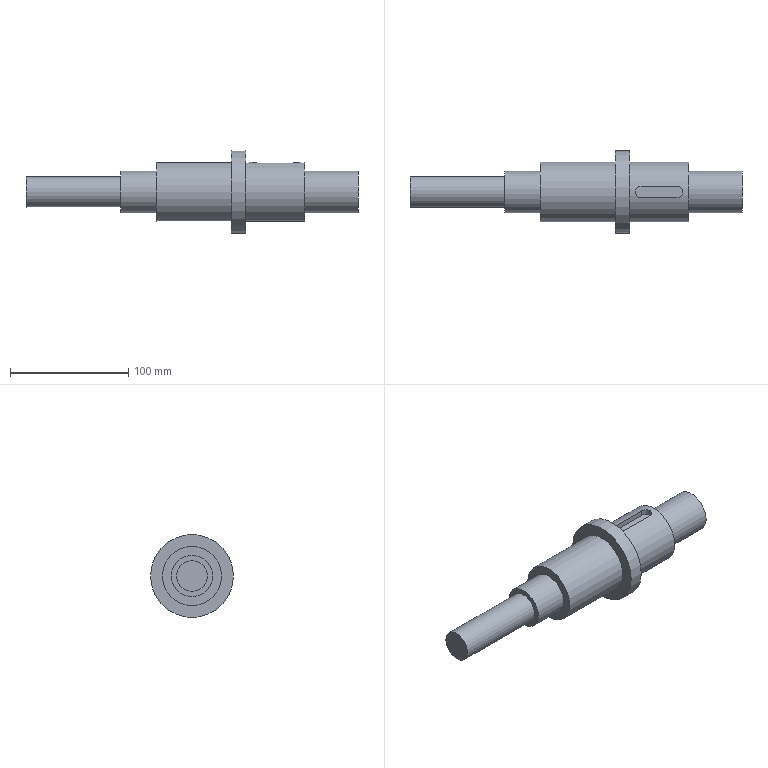Component | NX | SHUCHUZHOU | 1 solid | 18 faces | box 280.5 x 70 x 70 mm | volume 381839 mm3 | plane 10 | cylinder 8 | commonest cylinder face diameters 50 x2 35 x2 10 x2 70 x1 26 x1
STEP:
#1=CARTESIAN_POINT('',(0.,0.,0.));
#2=DIRECTION('',(0.,0.,1.));
#3=DIRECTION('',(1.,0.,0.));
#4=AXIS2_PLACEMENT_3D('',#1,#2,#3);
#5=CARTESIAN_POINT('',(5.25,225.,-88.));
#6=VERTEX_POINT('',#5);
#7=CARTESIAN_POINT('',(5.25,200.,-88.));
#8=DIRECTION('',(1.,0.,0.));
#9=DIRECTION('',(0.,1.,0.));
#10=AXIS2_PLACEMENT_3D('',#7,#8,#9);
#11=CIRCLE('',#10,25.);
#12=CARTESIAN_POINT('',(55.25,200.,-88.));
#13=DIRECTION('',(-1.,0.,0.));
#14=DIRECTION('',(0.,0.,1.));
#15=AXIS2_PLACEMENT_3D('',#12,#13,#14);
#16=CYLINDRICAL_SURFACE('',#15,25.);
#17=CARTESIAN_POINT('',(7.854,50.));
#18=DIRECTION('',(-1.,0.));
#19=VECTOR('',#18,1.);
#20=LINE('',#17,#19);
#21=(GEOMETRIC_REPRESENTATION_CONTEXT(2)PARAMETRIC_REPRESENTATION_CONTEXT()REPRESENTATION_CONTEXT('',''));
#22=DEFINITIONAL_REPRESENTATION('',(#20),#21);
#23=PCURVE('',#16,#22);
#24=CARTESIAN_POINT('',(5.25,200.,-88.));
#25=DIRECTION('',(1.,0.,0.));
#26=DIRECTION('',(0.,0.,-1.));
#27=AXIS2_PLACEMENT_3D('',#24,#25,#26);
#28=PLANE('',#27);
#29=CARTESIAN_POINT('',(0.,0.));
#30=DIRECTION('',(0.,1.));
#31=AXIS2_PLACEMENT_2D('',#29,#30);
#32=CIRCLE('',#31,25.);
#33=(GEOMETRIC_REPRESENTATION_CONTEXT(2)PARAMETRIC_REPRESENTATION_CONTEXT()REPRESENTATION_CONTEXT('',''));
#34=DEFINITIONAL_REPRESENTATION('',(#32),#33);
#35=PCURVE('',#28,#34);
#36=SURFACE_CURVE('',#11,(#23,#35),.PCURVE_S1.);
#37=EDGE_CURVE('',#6,#6,#36,.T.);
#38=ORIENTED_EDGE('',*,*,#37,.T.);
#39=CARTESIAN_POINT('',(55.25,225.,-88.));
#40=VERTEX_POINT('',#39);
#41=CARTESIAN_POINT('',(55.25,225.,-88.));
#42=CARTESIAN_POINT('',(5.25,225.,-88.));
#43=B_SPLINE_CURVE_WITH_KNOTS('',1,(#41,#42),.UNSPECIFIED.,.F.,.F.,(2,2),(0.,50.),.PIECEWISE_BEZIER_KNOTS.);
#44=CARTESIAN_POINT('',(1.571,0.));
#45=DIRECTION('',(0.,1.));
#46=VECTOR('',#45,1.);
#47=LINE('',#44,#46);
#48=(GEOMETRIC_REPRESENTATION_CONTEXT(2)PARAMETRIC_REPRESENTATION_CONTEXT()REPRESENTATION_CONTEXT('',''));
#49=DEFINITIONAL_REPRESENTATION('',(#47),#48);
#50=PCURVE('',#16,#49);
#51=CARTESIAN_POINT('',(7.854,0.));
#52=DIRECTION('',(0.,1.));
#53=VECTOR('',#52,1.);
#54=LINE('',#51,#53);
#55=(GEOMETRIC_REPRESENTATION_CONTEXT(2)PARAMETRIC_REPRESENTATION_CONTEXT()REPRESENTATION_CONTEXT('',''));
#56=DEFINITIONAL_REPRESENTATION('',(#54),#55);
#57=PCURVE('',#16,#56);
#58=SEAM_CURVE('',#43,(#50,#57),.PCURVE_S1.);
#59=EDGE_CURVE('',#40,#6,#58,.T.);
#60=ORIENTED_EDGE('',*,*,#59,.F.);
#61=CARTESIAN_POINT('',(55.25,200.,-88.));
#62=DIRECTION('',(1.,0.,0.));
#63=DIRECTION('',(0.,1.,0.));
#64=AXIS2_PLACEMENT_3D('',#61,#62,#63);
#65=CIRCLE('',#64,25.);
#66=CARTESIAN_POINT('',(7.854,0.));
#67=DIRECTION('',(-1.,0.));
#68=VECTOR('',#67,1.);
#69=LINE('',#66,#68);
#70=(GEOMETRIC_REPRESENTATION_CONTEXT(2)PARAMETRIC_REPRESENTATION_CONTEXT()REPRESENTATION_CONTEXT('',''));
#71=DEFINITIONAL_REPRESENTATION('',(#69),#70);
#72=PCURVE('',#16,#71);
#73=CARTESIAN_POINT('',(55.25,200.,-88.));
#74=DIRECTION('',(1.,0.,0.));
#75=DIRECTION('',(0.,0.,-1.));
#76=AXIS2_PLACEMENT_3D('',#73,#74,#75);
#77=PLANE('',#76);
#78=CARTESIAN_POINT('',(0.,0.));
#79=DIRECTION('',(0.,1.));
#80=AXIS2_PLACEMENT_2D('',#78,#79);
#81=CIRCLE('',#80,25.);
#82=(GEOMETRIC_REPRESENTATION_CONTEXT(2)PARAMETRIC_REPRESENTATION_CONTEXT()REPRESENTATION_CONTEXT('',''));
#83=DEFINITIONAL_REPRESENTATION('',(#81),#82);
#84=PCURVE('',#77,#83);
#85=SURFACE_CURVE('',#65,(#72,#84),.PCURVE_S1.);
#86=EDGE_CURVE('',#40,#40,#85,.T.);
#87=ORIENTED_EDGE('',*,*,#86,.F.);
#88=ORIENTED_EDGE('',*,*,#59,.T.);
#89=EDGE_LOOP('',(#38,#60,#87,#88));
#90=FACE_BOUND('',#89,.T.);
#91=CARTESIAN_POINT('',(15.25,205.,-63.505));
#92=VERTEX_POINT('',#91);
#93=CARTESIAN_POINT('',(15.25,195.,-63.505));
#94=VERTEX_POINT('',#93);
#95=CARTESIAN_POINT('',(15.25,205.,-63.505));
#96=CARTESIAN_POINT('',(13.925,205.,-63.505));
#97=CARTESIAN_POINT('',(12.634,204.455,-63.383));
#98=CARTESIAN_POINT('',(10.795,202.616,-63.12));
#99=CARTESIAN_POINT('',(10.251,201.312,-63.));
#100=CARTESIAN_POINT('',(10.249,198.696,-63.));
#101=CARTESIAN_POINT('',(10.784,197.396,-63.118));
#102=CARTESIAN_POINT('',(12.641,195.536,-63.384));
#103=CARTESIAN_POINT('',(13.925,195.,-63.505));
#104=CARTESIAN_POINT('',(15.25,195.,-63.505));
#105=B_SPLINE_CURVE_WITH_KNOTS('',3,(#95,#96,#97,#98,#99,#100,#101,#102,#103,#104),.UNSPECIFIED.,.F.,.F.,(4,2,2,2,4),(0.,0.25,0.5,0.75,1.),.UNSPECIFIED.);
#106=CARTESIAN_POINT('',(6.485,40.));
#107=CARTESIAN_POINT('',(6.485,40.241));
#108=CARTESIAN_POINT('',(6.483,40.72));
#109=CARTESIAN_POINT('',(6.477,41.421));
#110=CARTESIAN_POINT('',(6.466,42.09));
#111=CARTESIAN_POINT('',(6.453,42.716));
#112=CARTESIAN_POINT('',(6.435,43.287));
#113=CARTESIAN_POINT('',(6.415,43.79));
#114=CARTESIAN_POINT('',(6.392,44.215));
#115=CARTESIAN_POINT('',(6.367,44.556));
#116=CARTESIAN_POINT('',(6.34,44.808));
#117=CARTESIAN_POINT('',(6.312,44.964));
#118=CARTESIAN_POINT('',(6.283,45.018));
#119=CARTESIAN_POINT('',(6.255,44.965));
#120=CARTESIAN_POINT('',(6.227,44.811));
#121=CARTESIAN_POINT('',(6.2,44.562));
#122=CARTESIAN_POINT('',(6.175,44.221));
#123=CARTESIAN_POINT('',(6.152,43.794));
#124=CARTESIAN_POINT('',(6.131,43.286));
#125=CARTESIAN_POINT('',(6.114,42.713));
#126=CARTESIAN_POINT('',(6.1,42.087));
#127=CARTESIAN_POINT('',(6.09,41.419));
#128=CARTESIAN_POINT('',(6.083,40.72));
#129=CARTESIAN_POINT('',(6.082,40.241));
#130=CARTESIAN_POINT('',(6.082,40.));
#131=B_SPLINE_CURVE_WITH_KNOTS('',3,(#106,#107,#108,#109,#110,#111,#112,#113,#114,#115,#116,#117,#118,#119,#120,#121,#122,#123,#124,#125,#126,#127,#128,#129,#130),.UNSPECIFIED.,.F.,.F.,(4,1,1,1,1,1,1,1,1,1,1,1,1,1,1,1,1,1,1,1,1,1,4),(0.,0.04545,0.09091,0.1364,0.1818,0.2273,0.2727,0.3182,0.3636,0.4091,0.4545,0.5,0.5455,0.5909,0.6364,0.6818,0.7273,0.7727,0.8182,0.8636,0.9091,0.9545,1.),.QUASI_UNIFORM_KNOTS.);
#132=(GEOMETRIC_REPRESENTATION_CONTEXT(2)PARAMETRIC_REPRESENTATION_CONTEXT()REPRESENTATION_CONTEXT('',''));
#133=DEFINITIONAL_REPRESENTATION('',(#131),#132);
#134=PCURVE('',#16,#133);
#135=CARTESIAN_POINT('',(15.25,200.,-27.));
#136=DIRECTION('',(0.,0.,-1.));
#137=DIRECTION('',(-1.,0.,0.));
#138=AXIS2_PLACEMENT_3D('',#135,#136,#137);
#139=CYLINDRICAL_SURFACE('',#138,5.);
#140=CARTESIAN_POINT('',(1.571,36.505));
#141=CARTESIAN_POINT('',(1.523,36.505));
#142=CARTESIAN_POINT('',(1.427,36.497));
#143=CARTESIAN_POINT('',(1.284,36.465));
#144=CARTESIAN_POINT('',(1.141,36.416));
#145=CARTESIAN_POINT('',(0.9983,36.356));
#146=CARTESIAN_POINT('',(0.8563,36.287));
#147=CARTESIAN_POINT('',(0.7145,36.215));
#148=CARTESIAN_POINT('',(0.5722,36.147));
#149=CARTESIAN_POINT('',(0.4294,36.087));
#150=CARTESIAN_POINT('',(0.2863,36.04));
#151=CARTESIAN_POINT('',(0.1435,36.008));
#152=CARTESIAN_POINT('',(0.0007954,35.996));
#153=CARTESIAN_POINT('',(-0.1418,36.008));
#154=CARTESIAN_POINT('',(-0.2844,36.039));
#155=CARTESIAN_POINT('',(-0.4273,36.087));
#156=CARTESIAN_POINT('',(-0.5702,36.146));
#157=CARTESIAN_POINT('',(-0.7132,36.214));
#158=CARTESIAN_POINT('',(-0.8566,36.288));
#159=CARTESIAN_POINT('',(-0.9991,36.356));
#160=CARTESIAN_POINT('',(-1.141,36.417));
#161=CARTESIAN_POINT('',(-1.284,36.465));
#162=CARTESIAN_POINT('',(-1.427,36.497));
#163=CARTESIAN_POINT('',(-1.523,36.505));
#164=CARTESIAN_POINT('',(-1.571,36.505));
#165=B_SPLINE_CURVE_WITH_KNOTS('',3,(#140,#141,#142,#143,#144,#145,#146,#147,#148,#149,#150,#151,#152,#153,#154,#155,#156,#157,#158,#159,#160,#161,#162,#163,#164),.UNSPECIFIED.,.F.,.F.,(4,1,1,1,1,1,1,1,1,1,1,1,1,1,1,1,1,1,1,1,1,1,4),(0.,0.04545,0.09091,0.1364,0.1818,0.2273,0.2727,0.3182,0.3636,0.4091,0.4545,0.5,0.5455,0.5909,0.6364,0.6818,0.7273,0.7727,0.8182,0.8636,0.9091,0.9545,1.),.QUASI_UNIFORM_KNOTS.);
#166=(GEOMETRIC_REPRESENTATION_CONTEXT(2)PARAMETRIC_REPRESENTATION_CONTEXT()REPRESENTATION_CONTEXT('',''));
#167=DEFINITIONAL_REPRESENTATION('',(#165),#166);
#168=PCURVE('',#139,#167);
#169=SURFACE_CURVE('',#105,(#134,#168),.PCURVE_S1.);
#170=EDGE_CURVE('',#92,#94,#169,.T.);
#171=ORIENTED_EDGE('',*,*,#170,.F.);
#172=CARTESIAN_POINT('',(45.25,205.,-63.505));
#173=VERTEX_POINT('',#172);
#174=CARTESIAN_POINT('',(55.25,205.,-63.505));
#175=DIRECTION('',(-1.,0.,0.));
#176=VECTOR('',#175,1.);
#177=LINE('',#174,#176);
#178=CARTESIAN_POINT('',(6.485,0.));
#179=DIRECTION('',(0.,1.));
#180=VECTOR('',#179,1.);
#181=LINE('',#178,#180);
#182=(GEOMETRIC_REPRESENTATION_CONTEXT(2)PARAMETRIC_REPRESENTATION_CONTEXT()REPRESENTATION_CONTEXT('',''));
#183=DEFINITIONAL_REPRESENTATION('',(#181),#182);
#184=PCURVE('',#16,#183);
#185=CARTESIAN_POINT('',(45.25,205.,-27.));
#186=DIRECTION('',(0.,-1.,0.));
#187=DIRECTION('',(0.,0.,-1.));
#188=AXIS2_PLACEMENT_3D('',#185,#186,#187);
#189=PLANE('',#188);
#190=CARTESIAN_POINT('',(36.505,10.));
#191=DIRECTION('',(0.,-1.));
#192=VECTOR('',#191,1.);
#193=LINE('',#190,#192);
#194=(GEOMETRIC_REPRESENTATION_CONTEXT(2)PARAMETRIC_REPRESENTATION_CONTEXT()REPRESENTATION_CONTEXT('',''));
#195=DEFINITIONAL_REPRESENTATION('',(#193),#194);
#196=PCURVE('',#189,#195);
#197=SURFACE_CURVE('',#177,(#184,#196),.PCURVE_S1.);
#198=EDGE_CURVE('',#173,#92,#197,.T.);
#199=ORIENTED_EDGE('',*,*,#198,.F.);
#200=CARTESIAN_POINT('',(45.25,195.,-63.505));
#201=VERTEX_POINT('',#200);
#202=CARTESIAN_POINT('',(45.25,195.,-63.505));
#203=CARTESIAN_POINT('',(46.575,195.,-63.505));
#204=CARTESIAN_POINT('',(47.866,195.545,-63.383));
#205=CARTESIAN_POINT('',(49.705,197.384,-63.12));
#206=CARTESIAN_POINT('',(50.249,198.688,-63.));
#207=CARTESIAN_POINT('',(50.251,201.304,-63.));
#208=CARTESIAN_POINT('',(49.716,202.604,-63.118));
#209=CARTESIAN_POINT('',(47.859,204.464,-63.384));
#210=CARTESIAN_POINT('',(46.575,205.,-63.505));
#211=CARTESIAN_POINT('',(45.25,205.,-63.505));
#212=B_SPLINE_CURVE_WITH_KNOTS('',3,(#202,#203,#204,#205,#206,#207,#208,#209,#210,#211),.UNSPECIFIED.,.F.,.F.,(4,2,2,2,4),(0.,0.25,0.5,0.75,1.),.UNSPECIFIED.);
#213=CARTESIAN_POINT('',(6.082,10.));
#214=CARTESIAN_POINT('',(6.082,9.759));
#215=CARTESIAN_POINT('',(6.083,9.28));
#216=CARTESIAN_POINT('',(6.09,8.579));
#217=CARTESIAN_POINT('',(6.1,7.91));
#218=CARTESIAN_POINT('',(6.114,7.284));
#219=CARTESIAN_POINT('',(6.131,6.713));
#220=CARTESIAN_POINT('',(6.151,6.21));
#221=CARTESIAN_POINT('',(6.174,5.785));
#222=CARTESIAN_POINT('',(6.2,5.444));
#223=CARTESIAN_POINT('',(6.227,5.192));
#224=CARTESIAN_POINT('',(6.254,5.036));
#225=CARTESIAN_POINT('',(6.283,4.982));
#226=CARTESIAN_POINT('',(6.312,5.035));
#227=CARTESIAN_POINT('',(6.339,5.189));
#228=CARTESIAN_POINT('',(6.366,5.438));
#229=CARTESIAN_POINT('',(6.392,5.779));
#230=CARTESIAN_POINT('',(6.415,6.206));
#231=CARTESIAN_POINT('',(6.435,6.714));
#232=CARTESIAN_POINT('',(6.453,7.287));
#233=CARTESIAN_POINT('',(6.467,7.913));
#234=CARTESIAN_POINT('',(6.477,8.581));
#235=CARTESIAN_POINT('',(6.483,9.28));
#236=CARTESIAN_POINT('',(6.485,9.759));
#237=CARTESIAN_POINT('',(6.485,10.));
#238=B_SPLINE_CURVE_WITH_KNOTS('',3,(#213,#214,#215,#216,#217,#218,#219,#220,#221,#222,#223,#224,#225,#226,#227,#228,#229,#230,#231,#232,#233,#234,#235,#236,#237),.UNSPECIFIED.,.F.,.F.,(4,1,1,1,1,1,1,1,1,1,1,1,1,1,1,1,1,1,1,1,1,1,4),(0.,0.04545,0.09091,0.1364,0.1818,0.2273,0.2727,0.3182,0.3636,0.4091,0.4545,0.5,0.5455,0.5909,0.6364,0.6818,0.7273,0.7727,0.8182,0.8636,0.9091,0.9545,1.),.QUASI_UNIFORM_KNOTS.);
#239=(GEOMETRIC_REPRESENTATION_CONTEXT(2)PARAMETRIC_REPRESENTATION_CONTEXT()REPRESENTATION_CONTEXT('',''));
#240=DEFINITIONAL_REPRESENTATION('',(#238),#239);
#241=PCURVE('',#16,#240);
#242=CARTESIAN_POINT('',(45.25,200.,-27.));
#243=DIRECTION('',(0.,0.,-1.));
#244=DIRECTION('',(-1.,0.,0.));
#245=AXIS2_PLACEMENT_3D('',#242,#243,#244);
#246=CYLINDRICAL_SURFACE('',#245,5.);
#247=CARTESIAN_POINT('',(4.712,36.505));
#248=CARTESIAN_POINT('',(4.664,36.505));
#249=CARTESIAN_POINT('',(4.568,36.497));
#250=CARTESIAN_POINT('',(4.425,36.465));
#251=CARTESIAN_POINT('',(4.282,36.416));
#252=CARTESIAN_POINT('',(4.14,36.356));
#253=CARTESIAN_POINT('',(3.998,36.287));
#254=CARTESIAN_POINT('',(3.856,36.215));
#255=CARTESIAN_POINT('',(3.714,36.147));
#256=CARTESIAN_POINT('',(3.571,36.087));
#257=CARTESIAN_POINT('',(3.428,36.04));
#258=CARTESIAN_POINT('',(3.285,36.008));
#259=CARTESIAN_POINT('',(3.142,35.996));
#260=CARTESIAN_POINT('',(3.,36.008));
#261=CARTESIAN_POINT('',(2.857,36.039));
#262=CARTESIAN_POINT('',(2.714,36.087));
#263=CARTESIAN_POINT('',(2.571,36.146));
#264=CARTESIAN_POINT('',(2.428,36.214));
#265=CARTESIAN_POINT('',(2.285,36.288));
#266=CARTESIAN_POINT('',(2.142,36.356));
#267=CARTESIAN_POINT('',(2.,36.417));
#268=CARTESIAN_POINT('',(1.858,36.465));
#269=CARTESIAN_POINT('',(1.715,36.497));
#270=CARTESIAN_POINT('',(1.619,36.505));
#271=CARTESIAN_POINT('',(1.571,36.505));
#272=B_SPLINE_CURVE_WITH_KNOTS('',3,(#247,#248,#249,#250,#251,#252,#253,#254,#255,#256,#257,#258,#259,#260,#261,#262,#263,#264,#265,#266,#267,#268,#269,#270,#271),.UNSPECIFIED.,.F.,.F.,(4,1,1,1,1,1,1,1,1,1,1,1,1,1,1,1,1,1,1,1,1,1,4),(0.,0.04545,0.09091,0.1364,0.1818,0.2273,0.2727,0.3182,0.3636,0.4091,0.4545,0.5,0.5455,0.5909,0.6364,0.6818,0.7273,0.7727,0.8182,0.8636,0.9091,0.9545,1.),.QUASI_UNIFORM_KNOTS.);
#273=(GEOMETRIC_REPRESENTATION_CONTEXT(2)PARAMETRIC_REPRESENTATION_CONTEXT()REPRESENTATION_CONTEXT('',''));
#274=DEFINITIONAL_REPRESENTATION('',(#272),#273);
#275=PCURVE('',#246,#274);
#276=SURFACE_CURVE('',#212,(#241,#275),.PCURVE_S1.);
#277=EDGE_CURVE('',#201,#173,#276,.T.);
#278=ORIENTED_EDGE('',*,*,#277,.F.);
#279=CARTESIAN_POINT('',(55.25,195.,-63.505));
#280=DIRECTION('',(1.,0.,0.));
#281=VECTOR('',#280,1.);
#282=LINE('',#279,#281);
#283=CARTESIAN_POINT('',(6.082,0.));
#284=DIRECTION('',(0.,-1.));
#285=VECTOR('',#284,1.);
#286=LINE('',#283,#285);
#287=(GEOMETRIC_REPRESENTATION_CONTEXT(2)PARAMETRIC_REPRESENTATION_CONTEXT()REPRESENTATION_CONTEXT('',''));
#288=DEFINITIONAL_REPRESENTATION('',(#286),#287);
#289=PCURVE('',#16,#288);
#290=CARTESIAN_POINT('',(15.25,195.,-27.));
#291=DIRECTION('',(-0.,1.,0.));
#292=DIRECTION('',(-1.,-0.,0.));
#293=AXIS2_PLACEMENT_3D('',#290,#291,#292);
#294=PLANE('',#293);
#295=CARTESIAN_POINT('',(-40.,-36.505));
#296=DIRECTION('',(-1.,0.));
#297=VECTOR('',#296,1.);
#298=LINE('',#295,#297);
#299=(GEOMETRIC_REPRESENTATION_CONTEXT(2)PARAMETRIC_REPRESENTATION_CONTEXT()REPRESENTATION_CONTEXT('',''));
#300=DEFINITIONAL_REPRESENTATION('',(#298),#299);
#301=PCURVE('',#294,#300);
#302=SURFACE_CURVE('',#282,(#289,#301),.PCURVE_S1.);
#303=EDGE_CURVE('',#94,#201,#302,.T.);
#304=ORIENTED_EDGE('',*,*,#303,.F.);
#305=EDGE_LOOP('',(#171,#199,#278,#304));
#306=FACE_BOUND('',#305,.T.);
#307=ADVANCED_FACE('',(#90,#306),#16,.T.);
#308=CARTESIAN_POINT('',(-6.75,235.,-88.));
#309=VERTEX_POINT('',#308);
#310=CARTESIAN_POINT('',(-6.75,200.,-88.));
#311=DIRECTION('',(1.,0.,0.));
#312=DIRECTION('',(0.,1.,0.));
#313=AXIS2_PLACEMENT_3D('',#310,#311,#312);
#314=CIRCLE('',#313,35.);
#315=CARTESIAN_POINT('',(-6.75,200.,-88.));
#316=DIRECTION('',(1.,0.,0.));
#317=DIRECTION('',(0.,0.,-1.));
#318=AXIS2_PLACEMENT_3D('',#315,#316,#317);
#319=PLANE('',#318);
#320=CARTESIAN_POINT('',(0.,0.));
#321=DIRECTION('',(0.,1.));
#322=AXIS2_PLACEMENT_2D('',#320,#321);
#323=CIRCLE('',#322,35.);
#324=(GEOMETRIC_REPRESENTATION_CONTEXT(2)PARAMETRIC_REPRESENTATION_CONTEXT()REPRESENTATION_CONTEXT('',''));
#325=DEFINITIONAL_REPRESENTATION('',(#323),#324);
#326=PCURVE('',#319,#325);
#327=CARTESIAN_POINT('',(5.25,200.,-88.));
#328=DIRECTION('',(-1.,0.,0.));
#329=DIRECTION('',(0.,0.,1.));
#330=AXIS2_PLACEMENT_3D('',#327,#328,#329);
#331=CYLINDRICAL_SURFACE('',#330,35.);
#332=CARTESIAN_POINT('',(7.854,12.));
#333=DIRECTION('',(-1.,0.));
#334=VECTOR('',#333,1.);
#335=LINE('',#332,#334);
#336=(GEOMETRIC_REPRESENTATION_CONTEXT(2)PARAMETRIC_REPRESENTATION_CONTEXT()REPRESENTATION_CONTEXT('',''));
#337=DEFINITIONAL_REPRESENTATION('',(#335),#336);
#338=PCURVE('',#331,#337);
#339=SURFACE_CURVE('',#314,(#326,#338),.PCURVE_S1.);
#340=EDGE_CURVE('',#309,#309,#339,.T.);
#341=ORIENTED_EDGE('',*,*,#340,.F.);
#342=EDGE_LOOP('',(#341));
#343=FACE_BOUND('',#342,.T.);
#344=CARTESIAN_POINT('',(-6.75,225.,-88.));
#345=VERTEX_POINT('',#344);
#346=CARTESIAN_POINT('',(-6.75,200.,-88.));
#347=DIRECTION('',(-1.,0.,0.));
#348=DIRECTION('',(0.,1.,0.));
#349=AXIS2_PLACEMENT_3D('',#346,#347,#348);
#350=CIRCLE('',#349,25.);
#351=CARTESIAN_POINT('',(0.,25.));
#352=CARTESIAN_POINT('',(43.301,25.));
#353=CARTESIAN_POINT('',(21.651,-12.5));
#354=CARTESIAN_POINT('',(0.,-50.));
#355=CARTESIAN_POINT('',(-21.651,-12.5));
#356=CARTESIAN_POINT('',(-43.301,25.));
#357=CARTESIAN_POINT('',(0.,25.));
#358=(BOUNDED_CURVE()B_SPLINE_CURVE(2,(#351,#352,#353,#354,#355,#356,#357),.UNSPECIFIED.,.T.,.F.)B_SPLINE_CURVE_WITH_KNOTS((1,2,2,2,2,1),(-2.094,0.,2.094,4.189,6.283,8.378),.UNSPECIFIED.)CURVE()GEOMETRIC_REPRESENTATION_ITEM()RATIONAL_B_SPLINE_CURVE((1.,0.5,1.,0.5,1.,0.5,1.))REPRESENTATION_ITEM(''));
#359=(GEOMETRIC_REPRESENTATION_CONTEXT(2)PARAMETRIC_REPRESENTATION_CONTEXT()REPRESENTATION_CONTEXT('',''));
#360=DEFINITIONAL_REPRESENTATION('',(#358),#359);
#361=PCURVE('',#319,#360);
#362=CARTESIAN_POINT('',(-70.25,200.,-88.));
#363=DIRECTION('',(1.,0.,0.));
#364=DIRECTION('',(0.,0.,-1.));
#365=AXIS2_PLACEMENT_3D('',#362,#363,#364);
#366=CYLINDRICAL_SURFACE('',#365,25.);
#367=CARTESIAN_POINT('',(7.854,63.5));
#368=DIRECTION('',(-1.,0.));
#369=VECTOR('',#368,1.);
#370=LINE('',#367,#369);
#371=(GEOMETRIC_REPRESENTATION_CONTEXT(2)PARAMETRIC_REPRESENTATION_CONTEXT()REPRESENTATION_CONTEXT('',''));
#372=DEFINITIONAL_REPRESENTATION('',(#370),#371);
#373=PCURVE('',#366,#372);
#374=SURFACE_CURVE('',#350,(#361,#373),.PCURVE_S1.);
#375=EDGE_CURVE('',#345,#345,#374,.T.);
#376=ORIENTED_EDGE('',*,*,#375,.F.);
#377=EDGE_LOOP('',(#376));
#378=FACE_BOUND('',#377,.T.);
#379=ADVANCED_FACE('',(#343,#378),#319,.F.);
#380=CARTESIAN_POINT('',(5.25,235.,-88.));
#381=VERTEX_POINT('',#380);
#382=CARTESIAN_POINT('',(5.25,200.,-88.));
#383=DIRECTION('',(1.,0.,0.));
#384=DIRECTION('',(0.,1.,0.));
#385=AXIS2_PLACEMENT_3D('',#382,#383,#384);
#386=CIRCLE('',#385,35.);
#387=CARTESIAN_POINT('',(7.854,0.));
#388=DIRECTION('',(-1.,0.));
#389=VECTOR('',#388,1.);
#390=LINE('',#387,#389);
#391=(GEOMETRIC_REPRESENTATION_CONTEXT(2)PARAMETRIC_REPRESENTATION_CONTEXT()REPRESENTATION_CONTEXT('',''));
#392=DEFINITIONAL_REPRESENTATION('',(#390),#391);
#393=PCURVE('',#331,#392);
#394=CARTESIAN_POINT('',(0.,0.));
#395=DIRECTION('',(0.,1.));
#396=AXIS2_PLACEMENT_2D('',#394,#395);
#397=CIRCLE('',#396,35.);
#398=(GEOMETRIC_REPRESENTATION_CONTEXT(2)PARAMETRIC_REPRESENTATION_CONTEXT()REPRESENTATION_CONTEXT('',''));
#399=DEFINITIONAL_REPRESENTATION('',(#397),#398);
#400=PCURVE('',#28,#399);
#401=SURFACE_CURVE('',#386,(#393,#400),.PCURVE_S1.);
#402=EDGE_CURVE('',#381,#381,#401,.T.);
#403=ORIENTED_EDGE('',*,*,#402,.F.);
#404=CARTESIAN_POINT('',(5.25,235.,-88.));
#405=CARTESIAN_POINT('',(-6.75,235.,-88.));
#406=B_SPLINE_CURVE_WITH_KNOTS('',1,(#404,#405),.UNSPECIFIED.,.F.,.F.,(2,2),(0.,12.),.PIECEWISE_BEZIER_KNOTS.);
#407=CARTESIAN_POINT('',(7.854,0.));
#408=DIRECTION('',(0.,1.));
#409=VECTOR('',#408,1.);
#410=LINE('',#407,#409);
#411=(GEOMETRIC_REPRESENTATION_CONTEXT(2)PARAMETRIC_REPRESENTATION_CONTEXT()REPRESENTATION_CONTEXT('',''));
#412=DEFINITIONAL_REPRESENTATION('',(#410),#411);
#413=PCURVE('',#331,#412);
#414=CARTESIAN_POINT('',(1.571,0.));
#415=DIRECTION('',(0.,1.));
#416=VECTOR('',#415,1.);
#417=LINE('',#414,#416);
#418=(GEOMETRIC_REPRESENTATION_CONTEXT(2)PARAMETRIC_REPRESENTATION_CONTEXT()REPRESENTATION_CONTEXT('',''));
#419=DEFINITIONAL_REPRESENTATION('',(#417),#418);
#420=PCURVE('',#331,#419);
#421=SEAM_CURVE('',#406,(#413,#420),.PCURVE_S1.);
#422=EDGE_CURVE('',#381,#309,#421,.T.);
#423=ORIENTED_EDGE('',*,*,#422,.T.);
#424=ORIENTED_EDGE('',*,*,#340,.T.);
#425=ORIENTED_EDGE('',*,*,#422,.F.);
#426=EDGE_LOOP('',(#403,#423,#424,#425));
#427=FACE_BOUND('',#426,.T.);
#428=ADVANCED_FACE('',(#427),#331,.T.);
#429=ORIENTED_EDGE('',*,*,#37,.F.);
#430=EDGE_LOOP('',(#429));
#431=FACE_BOUND('',#430,.T.);
#432=ORIENTED_EDGE('',*,*,#402,.T.);
#433=EDGE_LOOP('',(#432));
#434=FACE_BOUND('',#433,.T.);
#435=ADVANCED_FACE('',(#431,#434),#28,.T.);
#436=CARTESIAN_POINT('',(55.25,217.5,-88.));
#437=VERTEX_POINT('',#436);
#438=CARTESIAN_POINT('',(55.25,200.,-88.));
#439=DIRECTION('',(1.,0.,0.));
#440=DIRECTION('',(0.,1.,0.));
#441=AXIS2_PLACEMENT_3D('',#438,#439,#440);
#442=CIRCLE('',#441,17.5);
#443=CARTESIAN_POINT('',(0.,0.));
#444=DIRECTION('',(0.,1.));
#445=AXIS2_PLACEMENT_2D('',#443,#444);
#446=CIRCLE('',#445,17.5);
#447=(GEOMETRIC_REPRESENTATION_CONTEXT(2)PARAMETRIC_REPRESENTATION_CONTEXT()REPRESENTATION_CONTEXT('',''));
#448=DEFINITIONAL_REPRESENTATION('',(#446),#447);
#449=PCURVE('',#77,#448);
#450=CARTESIAN_POINT('',(100.25,200.,-88.));
#451=DIRECTION('',(-1.,0.,0.));
#452=DIRECTION('',(0.,0.,1.));
#453=AXIS2_PLACEMENT_3D('',#450,#451,#452);
#454=CYLINDRICAL_SURFACE('',#453,17.5);
#455=CARTESIAN_POINT('',(7.854,45.));
#456=DIRECTION('',(-1.,0.));
#457=VECTOR('',#456,1.);
#458=LINE('',#455,#457);
#459=(GEOMETRIC_REPRESENTATION_CONTEXT(2)PARAMETRIC_REPRESENTATION_CONTEXT()REPRESENTATION_CONTEXT('',''));
#460=DEFINITIONAL_REPRESENTATION('',(#458),#459);
#461=PCURVE('',#454,#460);
#462=SURFACE_CURVE('',#442,(#449,#461),.PCURVE_S1.);
#463=EDGE_CURVE('',#437,#437,#462,.T.);
#464=ORIENTED_EDGE('',*,*,#463,.F.);
#465=EDGE_LOOP('',(#464));
#466=FACE_BOUND('',#465,.T.);
#467=ORIENTED_EDGE('',*,*,#86,.T.);
#468=EDGE_LOOP('',(#467));
#469=FACE_BOUND('',#468,.T.);
#470=ADVANCED_FACE('',(#466,#469),#77,.T.);
#471=CARTESIAN_POINT('',(100.25,217.5,-88.));
#472=VERTEX_POINT('',#471);
#473=CARTESIAN_POINT('',(100.25,200.,-88.));
#474=DIRECTION('',(1.,0.,0.));
#475=DIRECTION('',(0.,1.,0.));
#476=AXIS2_PLACEMENT_3D('',#473,#474,#475);
#477=CIRCLE('',#476,17.5);
#478=CARTESIAN_POINT('',(7.854,0.));
#479=DIRECTION('',(-1.,0.));
#480=VECTOR('',#479,1.);
#481=LINE('',#478,#480);
#482=(GEOMETRIC_REPRESENTATION_CONTEXT(2)PARAMETRIC_REPRESENTATION_CONTEXT()REPRESENTATION_CONTEXT('',''));
#483=DEFINITIONAL_REPRESENTATION('',(#481),#482);
#484=PCURVE('',#454,#483);
#485=CARTESIAN_POINT('',(100.25,200.,-88.));
#486=DIRECTION('',(1.,0.,0.));
#487=DIRECTION('',(0.,0.,-1.));
#488=AXIS2_PLACEMENT_3D('',#485,#486,#487);
#489=PLANE('',#488);
#490=CARTESIAN_POINT('',(0.,0.));
#491=DIRECTION('',(0.,1.));
#492=AXIS2_PLACEMENT_2D('',#490,#491);
#493=CIRCLE('',#492,17.5);
#494=(GEOMETRIC_REPRESENTATION_CONTEXT(2)PARAMETRIC_REPRESENTATION_CONTEXT()REPRESENTATION_CONTEXT('',''));
#495=DEFINITIONAL_REPRESENTATION('',(#493),#494);
#496=PCURVE('',#489,#495);
#497=SURFACE_CURVE('',#477,(#484,#496),.PCURVE_S1.);
#498=EDGE_CURVE('',#472,#472,#497,.T.);
#499=ORIENTED_EDGE('',*,*,#498,.F.);
#500=CARTESIAN_POINT('',(100.25,217.5,-88.));
#501=CARTESIAN_POINT('',(55.25,217.5,-88.));
#502=B_SPLINE_CURVE_WITH_KNOTS('',1,(#500,#501),.UNSPECIFIED.,.F.,.F.,(2,2),(0.,45.),.PIECEWISE_BEZIER_KNOTS.);
#503=CARTESIAN_POINT('',(7.854,0.));
#504=DIRECTION('',(0.,1.));
#505=VECTOR('',#504,1.);
#506=LINE('',#503,#505);
#507=(GEOMETRIC_REPRESENTATION_CONTEXT(2)PARAMETRIC_REPRESENTATION_CONTEXT()REPRESENTATION_CONTEXT('',''));
#508=DEFINITIONAL_REPRESENTATION('',(#506),#507);
#509=PCURVE('',#454,#508);
#510=CARTESIAN_POINT('',(1.571,0.));
#511=DIRECTION('',(0.,1.));
#512=VECTOR('',#511,1.);
#513=LINE('',#510,#512);
#514=(GEOMETRIC_REPRESENTATION_CONTEXT(2)PARAMETRIC_REPRESENTATION_CONTEXT()REPRESENTATION_CONTEXT('',''));
#515=DEFINITIONAL_REPRESENTATION('',(#513),#514);
#516=PCURVE('',#454,#515);
#517=SEAM_CURVE('',#502,(#509,#516),.PCURVE_S1.);
#518=EDGE_CURVE('',#472,#437,#517,.T.);
#519=ORIENTED_EDGE('',*,*,#518,.T.);
#520=ORIENTED_EDGE('',*,*,#463,.T.);
#521=ORIENTED_EDGE('',*,*,#518,.F.);
#522=EDGE_LOOP('',(#499,#519,#520,#521));
#523=FACE_BOUND('',#522,.T.);
#524=ADVANCED_FACE('',(#523),#454,.T.);
#525=ORIENTED_EDGE('',*,*,#498,.T.);
#526=EDGE_LOOP('',(#525));
#527=FACE_BOUND('',#526,.T.);
#528=ADVANCED_FACE('',(#527),#489,.T.);
#529=CARTESIAN_POINT('',(-70.25,225.,-88.));
#530=VERTEX_POINT('',#529);
#531=CARTESIAN_POINT('',(-70.25,200.,-88.));
#532=DIRECTION('',(-1.,0.,0.));
#533=DIRECTION('',(0.,1.,0.));
#534=AXIS2_PLACEMENT_3D('',#531,#532,#533);
#535=CIRCLE('',#534,25.);
#536=CARTESIAN_POINT('',(7.854,0.));
#537=DIRECTION('',(-1.,0.));
#538=VECTOR('',#537,1.);
#539=LINE('',#536,#538);
#540=(GEOMETRIC_REPRESENTATION_CONTEXT(2)PARAMETRIC_REPRESENTATION_CONTEXT()REPRESENTATION_CONTEXT('',''));
#541=DEFINITIONAL_REPRESENTATION('',(#539),#540);
#542=PCURVE('',#366,#541);
#543=CARTESIAN_POINT('',(-70.25,200.,-88.));
#544=DIRECTION('',(-1.,0.,0.));
#545=DIRECTION('',(0.,0.,1.));
#546=AXIS2_PLACEMENT_3D('',#543,#544,#545);
#547=PLANE('',#546);
#548=CARTESIAN_POINT('',(0.,0.));
#549=DIRECTION('',(0.,1.));
#550=AXIS2_PLACEMENT_2D('',#548,#549);
#551=CIRCLE('',#550,25.);
#552=(GEOMETRIC_REPRESENTATION_CONTEXT(2)PARAMETRIC_REPRESENTATION_CONTEXT()REPRESENTATION_CONTEXT('',''));
#553=DEFINITIONAL_REPRESENTATION('',(#551),#552);
#554=PCURVE('',#547,#553);
#555=SURFACE_CURVE('',#535,(#542,#554),.PCURVE_S1.);
#556=EDGE_CURVE('',#530,#530,#555,.T.);
#557=ORIENTED_EDGE('',*,*,#556,.F.);
#558=CARTESIAN_POINT('',(-70.25,225.,-88.));
#559=CARTESIAN_POINT('',(-6.75,225.,-88.));
#560=B_SPLINE_CURVE_WITH_KNOTS('',1,(#558,#559),.UNSPECIFIED.,.F.,.F.,(2,2),(0.,63.5),.PIECEWISE_BEZIER_KNOTS.);
#561=CARTESIAN_POINT('',(7.854,0.));
#562=DIRECTION('',(0.,1.));
#563=VECTOR('',#562,1.);
#564=LINE('',#561,#563);
#565=(GEOMETRIC_REPRESENTATION_CONTEXT(2)PARAMETRIC_REPRESENTATION_CONTEXT()REPRESENTATION_CONTEXT('',''));
#566=DEFINITIONAL_REPRESENTATION('',(#564),#565);
#567=PCURVE('',#366,#566);
#568=CARTESIAN_POINT('',(1.571,0.));
#569=DIRECTION('',(0.,1.));
#570=VECTOR('',#569,1.);
#571=LINE('',#568,#570);
#572=(GEOMETRIC_REPRESENTATION_CONTEXT(2)PARAMETRIC_REPRESENTATION_CONTEXT()REPRESENTATION_CONTEXT('',''));
#573=DEFINITIONAL_REPRESENTATION('',(#571),#572);
#574=PCURVE('',#366,#573);
#575=SEAM_CURVE('',#560,(#567,#574),.PCURVE_S1.);
#576=EDGE_CURVE('',#530,#345,#575,.T.);
#577=ORIENTED_EDGE('',*,*,#576,.T.);
#578=ORIENTED_EDGE('',*,*,#375,.T.);
#579=ORIENTED_EDGE('',*,*,#576,.F.);
#580=EDGE_LOOP('',(#557,#577,#578,#579));
#581=FACE_BOUND('',#580,.T.);
#582=ADVANCED_FACE('',(#581),#366,.T.);
#583=CARTESIAN_POINT('',(-70.25,217.5,-88.));
#584=VERTEX_POINT('',#583);
#585=CARTESIAN_POINT('',(-70.25,200.,-88.));
#586=DIRECTION('',(-1.,0.,0.));
#587=DIRECTION('',(0.,1.,0.));
#588=AXIS2_PLACEMENT_3D('',#585,#586,#587);
#589=CIRCLE('',#588,17.5);
#590=CARTESIAN_POINT('',(0.,0.));
#591=DIRECTION('',(0.,1.));
#592=AXIS2_PLACEMENT_2D('',#590,#591);
#593=CIRCLE('',#592,17.5);
#594=(GEOMETRIC_REPRESENTATION_CONTEXT(2)PARAMETRIC_REPRESENTATION_CONTEXT()REPRESENTATION_CONTEXT('',''));
#595=DEFINITIONAL_REPRESENTATION('',(#593),#594);
#596=PCURVE('',#547,#595);
#597=CARTESIAN_POINT('',(-100.25,200.,-88.));
#598=DIRECTION('',(1.,0.,0.));
#599=DIRECTION('',(0.,0.,-1.));
#600=AXIS2_PLACEMENT_3D('',#597,#598,#599);
#601=CYLINDRICAL_SURFACE('',#600,17.5);
#602=CARTESIAN_POINT('',(7.854,30.));
#603=DIRECTION('',(-1.,0.));
#604=VECTOR('',#603,1.);
#605=LINE('',#602,#604);
#606=(GEOMETRIC_REPRESENTATION_CONTEXT(2)PARAMETRIC_REPRESENTATION_CONTEXT()REPRESENTATION_CONTEXT('',''));
#607=DEFINITIONAL_REPRESENTATION('',(#605),#606);
#608=PCURVE('',#601,#607);
#609=SURFACE_CURVE('',#589,(#596,#608),.PCURVE_S1.);
#610=EDGE_CURVE('',#584,#584,#609,.T.);
#611=ORIENTED_EDGE('',*,*,#610,.F.);
#612=EDGE_LOOP('',(#611));
#613=FACE_BOUND('',#612,.T.);
#614=ORIENTED_EDGE('',*,*,#556,.T.);
#615=EDGE_LOOP('',(#614));
#616=FACE_BOUND('',#615,.T.);
#617=ADVANCED_FACE('',(#613,#616),#547,.T.);
#618=CARTESIAN_POINT('',(-100.25,217.5,-88.));
#619=VERTEX_POINT('',#618);
#620=CARTESIAN_POINT('',(-100.25,200.,-88.));
#621=DIRECTION('',(-1.,0.,0.));
#622=DIRECTION('',(0.,1.,0.));
#623=AXIS2_PLACEMENT_3D('',#620,#621,#622);
#624=CIRCLE('',#623,17.5);
#625=CARTESIAN_POINT('',(7.854,0.));
#626=DIRECTION('',(-1.,0.));
#627=VECTOR('',#626,1.);
#628=LINE('',#625,#627);
#629=(GEOMETRIC_REPRESENTATION_CONTEXT(2)PARAMETRIC_REPRESENTATION_CONTEXT()REPRESENTATION_CONTEXT('',''));
#630=DEFINITIONAL_REPRESENTATION('',(#628),#629);
#631=PCURVE('',#601,#630);
#632=CARTESIAN_POINT('',(-100.25,200.,-88.));
#633=DIRECTION('',(-1.,0.,0.));
#634=DIRECTION('',(0.,0.,1.));
#635=AXIS2_PLACEMENT_3D('',#632,#633,#634);
#636=PLANE('',#635);
#637=CARTESIAN_POINT('',(0.,0.));
#638=DIRECTION('',(0.,1.));
#639=AXIS2_PLACEMENT_2D('',#637,#638);
#640=CIRCLE('',#639,17.5);
#641=(GEOMETRIC_REPRESENTATION_CONTEXT(2)PARAMETRIC_REPRESENTATION_CONTEXT()REPRESENTATION_CONTEXT('',''));
#642=DEFINITIONAL_REPRESENTATION('',(#640),#641);
#643=PCURVE('',#636,#642);
#644=SURFACE_CURVE('',#624,(#631,#643),.PCURVE_S1.);
#645=EDGE_CURVE('',#619,#619,#644,.T.);
#646=ORIENTED_EDGE('',*,*,#645,.F.);
#647=CARTESIAN_POINT('',(-100.25,217.5,-88.));
#648=CARTESIAN_POINT('',(-70.25,217.5,-88.));
#649=B_SPLINE_CURVE_WITH_KNOTS('',1,(#647,#648),.UNSPECIFIED.,.F.,.F.,(2,2),(0.,30.),.PIECEWISE_BEZIER_KNOTS.);
#650=CARTESIAN_POINT('',(7.854,0.));
#651=DIRECTION('',(0.,1.));
#652=VECTOR('',#651,1.);
#653=LINE('',#650,#652);
#654=(GEOMETRIC_REPRESENTATION_CONTEXT(2)PARAMETRIC_REPRESENTATION_CONTEXT()REPRESENTATION_CONTEXT('',''));
#655=DEFINITIONAL_REPRESENTATION('',(#653),#654);
#656=PCURVE('',#601,#655);
#657=CARTESIAN_POINT('',(1.571,0.));
#658=DIRECTION('',(0.,1.));
#659=VECTOR('',#658,1.);
#660=LINE('',#657,#659);
#661=(GEOMETRIC_REPRESENTATION_CONTEXT(2)PARAMETRIC_REPRESENTATION_CONTEXT()REPRESENTATION_CONTEXT('',''));
#662=DEFINITIONAL_REPRESENTATION('',(#660),#661);
#663=PCURVE('',#601,#662);
#664=SEAM_CURVE('',#649,(#656,#663),.PCURVE_S1.);
#665=EDGE_CURVE('',#619,#584,#664,.T.);
#666=ORIENTED_EDGE('',*,*,#665,.T.);
#667=ORIENTED_EDGE('',*,*,#610,.T.);
#668=ORIENTED_EDGE('',*,*,#665,.F.);
#669=EDGE_LOOP('',(#646,#666,#667,#668));
#670=FACE_BOUND('',#669,.T.);
#671=ADVANCED_FACE('',(#670),#601,.T.);
#672=CARTESIAN_POINT('',(-100.25,213.,-88.));
#673=VERTEX_POINT('',#672);
#674=CARTESIAN_POINT('',(-100.25,200.,-88.));
#675=DIRECTION('',(-1.,0.,0.));
#676=DIRECTION('',(0.,1.,0.));
#677=AXIS2_PLACEMENT_3D('',#674,#675,#676);
#678=CIRCLE('',#677,13.);
#679=CARTESIAN_POINT('',(0.,0.));
#680=DIRECTION('',(0.,1.));
#681=AXIS2_PLACEMENT_2D('',#679,#680);
#682=CIRCLE('',#681,13.);
#683=(GEOMETRIC_REPRESENTATION_CONTEXT(2)PARAMETRIC_REPRESENTATION_CONTEXT()REPRESENTATION_CONTEXT('',''));
#684=DEFINITIONAL_REPRESENTATION('',(#682),#683);
#685=PCURVE('',#636,#684);
#686=CARTESIAN_POINT('',(-180.25,200.,-88.));
#687=DIRECTION('',(1.,0.,0.));
#688=DIRECTION('',(0.,0.,-1.));
#689=AXIS2_PLACEMENT_3D('',#686,#687,#688);
#690=CYLINDRICAL_SURFACE('',#689,13.);
#691=CARTESIAN_POINT('',(7.854,80.));
#692=DIRECTION('',(-1.,0.));
#693=VECTOR('',#692,1.);
#694=LINE('',#691,#693);
#695=(GEOMETRIC_REPRESENTATION_CONTEXT(2)PARAMETRIC_REPRESENTATION_CONTEXT()REPRESENTATION_CONTEXT('',''));
#696=DEFINITIONAL_REPRESENTATION('',(#694),#695);
#697=PCURVE('',#690,#696);
#698=SURFACE_CURVE('',#678,(#685,#697),.PCURVE_S1.);
#699=EDGE_CURVE('',#673,#673,#698,.T.);
#700=ORIENTED_EDGE('',*,*,#699,.F.);
#701=EDGE_LOOP('',(#700));
#702=FACE_BOUND('',#701,.T.);
#703=ORIENTED_EDGE('',*,*,#645,.T.);
#704=EDGE_LOOP('',(#703));
#705=FACE_BOUND('',#704,.T.);
#706=ADVANCED_FACE('',(#702,#705),#636,.T.);
#707=CARTESIAN_POINT('',(15.25,205.,-68.));
#708=VERTEX_POINT('',#707);
#709=CARTESIAN_POINT('',(15.25,205.,-27.));
#710=DIRECTION('',(0.,0.,1.));
#711=VECTOR('',#710,1.);
#712=LINE('',#709,#711);
#713=CARTESIAN_POINT('',(1.571,0.));
#714=DIRECTION('',(0.,-1.));
#715=VECTOR('',#714,1.);
#716=LINE('',#713,#715);
#717=(GEOMETRIC_REPRESENTATION_CONTEXT(2)PARAMETRIC_REPRESENTATION_CONTEXT()REPRESENTATION_CONTEXT('',''));
#718=DEFINITIONAL_REPRESENTATION('',(#716),#717);
#719=PCURVE('',#139,#718);
#720=CARTESIAN_POINT('',(0.,-30.));
#721=DIRECTION('',(-1.,0.));
#722=VECTOR('',#721,1.);
#723=LINE('',#720,#722);
#724=(GEOMETRIC_REPRESENTATION_CONTEXT(2)PARAMETRIC_REPRESENTATION_CONTEXT()REPRESENTATION_CONTEXT('',''));
#725=DEFINITIONAL_REPRESENTATION('',(#723),#724);
#726=PCURVE('',#189,#725);
#727=SURFACE_CURVE('',#712,(#719,#726),.PCURVE_S1.);
#728=EDGE_CURVE('',#708,#92,#727,.T.);
#729=ORIENTED_EDGE('',*,*,#728,.F.);
#730=CARTESIAN_POINT('',(15.25,195.,-68.));
#731=VERTEX_POINT('',#730);
#732=CARTESIAN_POINT('',(15.25,200.,-68.));
#733=DIRECTION('',(0.,0.,-1.));
#734=DIRECTION('',(1.,0.,0.));
#735=AXIS2_PLACEMENT_3D('',#732,#733,#734);
#736=CIRCLE('',#735,5.);
#737=CARTESIAN_POINT('',(-3.142,41.));
#738=DIRECTION('',(1.,0.));
#739=VECTOR('',#738,1.);
#740=LINE('',#737,#739);
#741=(GEOMETRIC_REPRESENTATION_CONTEXT(2)PARAMETRIC_REPRESENTATION_CONTEXT()REPRESENTATION_CONTEXT('',''));
#742=DEFINITIONAL_REPRESENTATION('',(#740),#741);
#743=PCURVE('',#139,#742);
#744=CARTESIAN_POINT('',(15.25,200.,-68.));
#745=DIRECTION('',(0.,0.,1.));
#746=DIRECTION('',(1.,0.,0.));
#747=AXIS2_PLACEMENT_3D('',#744,#745,#746);
#748=PLANE('',#747);
#749=CARTESIAN_POINT('',(5.,0.));
#750=CARTESIAN_POINT('',(5.,-8.66));
#751=CARTESIAN_POINT('',(-2.5,-4.33));
#752=CARTESIAN_POINT('',(-10.,-0.));
#753=CARTESIAN_POINT('',(-2.5,4.33));
#754=CARTESIAN_POINT('',(5.,8.66));
#755=CARTESIAN_POINT('',(5.,0.));
#756=(BOUNDED_CURVE()B_SPLINE_CURVE(2,(#749,#750,#751,#752,#753,#754,#755),.UNSPECIFIED.,.T.,.F.)B_SPLINE_CURVE_WITH_KNOTS((1,2,2,2,2,1),(-2.094,0.,2.094,4.189,6.283,8.378),.UNSPECIFIED.)CURVE()GEOMETRIC_REPRESENTATION_ITEM()RATIONAL_B_SPLINE_CURVE((1.,0.5,1.,0.5,1.,0.5,1.))REPRESENTATION_ITEM(''));
#757=(GEOMETRIC_REPRESENTATION_CONTEXT(2)PARAMETRIC_REPRESENTATION_CONTEXT()REPRESENTATION_CONTEXT('',''));
#758=DEFINITIONAL_REPRESENTATION('',(#756),#757);
#759=PCURVE('',#748,#758);
#760=SURFACE_CURVE('',#736,(#743,#759),.PCURVE_S1.);
#761=EDGE_CURVE('',#731,#708,#760,.T.);
#762=ORIENTED_EDGE('',*,*,#761,.F.);
#763=CARTESIAN_POINT('',(15.25,195.,-27.));
#764=DIRECTION('',(0.,0.,1.));
#765=VECTOR('',#764,1.);
#766=LINE('',#763,#765);
#767=CARTESIAN_POINT('',(-1.571,0.));
#768=DIRECTION('',(0.,-1.));
#769=VECTOR('',#768,1.);
#770=LINE('',#767,#769);
#771=(GEOMETRIC_REPRESENTATION_CONTEXT(2)PARAMETRIC_REPRESENTATION_CONTEXT()REPRESENTATION_CONTEXT('',''));
#772=DEFINITIONAL_REPRESENTATION('',(#770),#771);
#773=PCURVE('',#139,#772);
#774=CARTESIAN_POINT('',(0.,0.));
#775=DIRECTION('',(0.,1.));
#776=VECTOR('',#775,1.);
#777=LINE('',#774,#776);
#778=(GEOMETRIC_REPRESENTATION_CONTEXT(2)PARAMETRIC_REPRESENTATION_CONTEXT()REPRESENTATION_CONTEXT('',''));
#779=DEFINITIONAL_REPRESENTATION('',(#777),#778);
#780=PCURVE('',#294,#779);
#781=SURFACE_CURVE('',#766,(#773,#780),.PCURVE_S1.);
#782=EDGE_CURVE('',#731,#94,#781,.T.);
#783=ORIENTED_EDGE('',*,*,#782,.T.);
#784=ORIENTED_EDGE('',*,*,#170,.F.);
#785=EDGE_LOOP('',(#729,#762,#783,#784));
#786=FACE_BOUND('',#785,.F.);
#787=ADVANCED_FACE('',(#786),#139,.F.);
#788=ORIENTED_EDGE('',*,*,#303,.T.);
#789=CARTESIAN_POINT('',(45.25,195.,-68.));
#790=VERTEX_POINT('',#789);
#791=CARTESIAN_POINT('',(45.25,195.,-27.));
#792=DIRECTION('',(0.,0.,1.));
#793=VECTOR('',#792,1.);
#794=LINE('',#791,#793);
#795=CARTESIAN_POINT('',(-30.,0.));
#796=DIRECTION('',(0.,1.));
#797=VECTOR('',#796,1.);
#798=LINE('',#795,#797);
#799=(GEOMETRIC_REPRESENTATION_CONTEXT(2)PARAMETRIC_REPRESENTATION_CONTEXT()REPRESENTATION_CONTEXT('',''));
#800=DEFINITIONAL_REPRESENTATION('',(#798),#799);
#801=PCURVE('',#294,#800);
#802=CARTESIAN_POINT('',(4.712,0.));
#803=DIRECTION('',(0.,-1.));
#804=VECTOR('',#803,1.);
#805=LINE('',#802,#804);
#806=(GEOMETRIC_REPRESENTATION_CONTEXT(2)PARAMETRIC_REPRESENTATION_CONTEXT()REPRESENTATION_CONTEXT('',''));
#807=DEFINITIONAL_REPRESENTATION('',(#805),#806);
#808=PCURVE('',#246,#807);
#809=SURFACE_CURVE('',#794,(#801,#808),.PCURVE_S1.);
#810=EDGE_CURVE('',#790,#201,#809,.T.);
#811=ORIENTED_EDGE('',*,*,#810,.F.);
#812=CARTESIAN_POINT('',(15.25,195.,-68.));
#813=DIRECTION('',(-1.,-0.,0.));
#814=VECTOR('',#813,1.);
#815=LINE('',#812,#814);
#816=CARTESIAN_POINT('',(0.,-41.));
#817=DIRECTION('',(1.,0.));
#818=VECTOR('',#817,1.);
#819=LINE('',#816,#818);
#820=(GEOMETRIC_REPRESENTATION_CONTEXT(2)PARAMETRIC_REPRESENTATION_CONTEXT()REPRESENTATION_CONTEXT('',''));
#821=DEFINITIONAL_REPRESENTATION('',(#819),#820);
#822=PCURVE('',#294,#821);
#823=CARTESIAN_POINT('',(0.,-5.));
#824=DIRECTION('',(-1.,-0.));
#825=VECTOR('',#824,1.);
#826=LINE('',#823,#825);
#827=(GEOMETRIC_REPRESENTATION_CONTEXT(2)PARAMETRIC_REPRESENTATION_CONTEXT()REPRESENTATION_CONTEXT('',''));
#828=DEFINITIONAL_REPRESENTATION('',(#826),#827);
#829=PCURVE('',#748,#828);
#830=SURFACE_CURVE('',#815,(#822,#829),.PCURVE_S1.);
#831=EDGE_CURVE('',#790,#731,#830,.T.);
#832=ORIENTED_EDGE('',*,*,#831,.T.);
#833=ORIENTED_EDGE('',*,*,#782,.T.);
#834=EDGE_LOOP('',(#788,#811,#832,#833));
#835=FACE_BOUND('',#834,.T.);
#836=ADVANCED_FACE('',(#835),#294,.T.);
#837=ORIENTED_EDGE('',*,*,#810,.F.);
#838=CARTESIAN_POINT('',(45.25,205.,-68.));
#839=VERTEX_POINT('',#838);
#840=CARTESIAN_POINT('',(45.25,200.,-68.));
#841=DIRECTION('',(0.,0.,-1.));
#842=DIRECTION('',(1.,0.,0.));
#843=AXIS2_PLACEMENT_3D('',#840,#841,#842);
#844=CIRCLE('',#843,5.);
#845=CARTESIAN_POINT('',(-3.142,41.));
#846=DIRECTION('',(1.,0.));
#847=VECTOR('',#846,1.);
#848=LINE('',#845,#847);
#849=(GEOMETRIC_REPRESENTATION_CONTEXT(2)PARAMETRIC_REPRESENTATION_CONTEXT()REPRESENTATION_CONTEXT('',''));
#850=DEFINITIONAL_REPRESENTATION('',(#848),#849);
#851=PCURVE('',#246,#850);
#852=CARTESIAN_POINT('',(35.,0.));
#853=CARTESIAN_POINT('',(35.,-8.66));
#854=CARTESIAN_POINT('',(27.5,-4.33));
#855=CARTESIAN_POINT('',(20.,-0.));
#856=CARTESIAN_POINT('',(27.5,4.33));
#857=CARTESIAN_POINT('',(35.,8.66));
#858=CARTESIAN_POINT('',(35.,0.));
#859=(BOUNDED_CURVE()B_SPLINE_CURVE(2,(#852,#853,#854,#855,#856,#857,#858),.UNSPECIFIED.,.T.,.F.)B_SPLINE_CURVE_WITH_KNOTS((1,2,2,2,2,1),(-2.094,0.,2.094,4.189,6.283,8.378),.UNSPECIFIED.)CURVE()GEOMETRIC_REPRESENTATION_ITEM()RATIONAL_B_SPLINE_CURVE((1.,0.5,1.,0.5,1.,0.5,1.))REPRESENTATION_ITEM(''));
#860=(GEOMETRIC_REPRESENTATION_CONTEXT(2)PARAMETRIC_REPRESENTATION_CONTEXT()REPRESENTATION_CONTEXT('',''));
#861=DEFINITIONAL_REPRESENTATION('',(#859),#860);
#862=PCURVE('',#748,#861);
#863=SURFACE_CURVE('',#844,(#851,#862),.PCURVE_S1.);
#864=EDGE_CURVE('',#839,#790,#863,.T.);
#865=ORIENTED_EDGE('',*,*,#864,.F.);
#866=CARTESIAN_POINT('',(45.25,205.,-27.));
#867=DIRECTION('',(0.,0.,1.));
#868=VECTOR('',#867,1.);
#869=LINE('',#866,#868);
#870=CARTESIAN_POINT('',(1.571,0.));
#871=DIRECTION('',(0.,-1.));
#872=VECTOR('',#871,1.);
#873=LINE('',#870,#872);
#874=(GEOMETRIC_REPRESENTATION_CONTEXT(2)PARAMETRIC_REPRESENTATION_CONTEXT()REPRESENTATION_CONTEXT('',''));
#875=DEFINITIONAL_REPRESENTATION('',(#873),#874);
#876=PCURVE('',#246,#875);
#877=CARTESIAN_POINT('',(0.,0.));
#878=DIRECTION('',(-1.,0.));
#879=VECTOR('',#878,1.);
#880=LINE('',#877,#879);
#881=(GEOMETRIC_REPRESENTATION_CONTEXT(2)PARAMETRIC_REPRESENTATION_CONTEXT()REPRESENTATION_CONTEXT('',''));
#882=DEFINITIONAL_REPRESENTATION('',(#880),#881);
#883=PCURVE('',#189,#882);
#884=SURFACE_CURVE('',#869,(#876,#883),.PCURVE_S1.);
#885=EDGE_CURVE('',#839,#173,#884,.T.);
#886=ORIENTED_EDGE('',*,*,#885,.T.);
#887=ORIENTED_EDGE('',*,*,#277,.F.);
#888=EDGE_LOOP('',(#837,#865,#886,#887));
#889=FACE_BOUND('',#888,.F.);
#890=ADVANCED_FACE('',(#889),#246,.F.);
#891=ORIENTED_EDGE('',*,*,#198,.T.);
#892=ORIENTED_EDGE('',*,*,#728,.F.);
#893=CARTESIAN_POINT('',(45.25,205.,-68.));
#894=DIRECTION('',(1.,0.,0.));
#895=VECTOR('',#894,1.);
#896=LINE('',#893,#895);
#897=CARTESIAN_POINT('',(41.,0.));
#898=DIRECTION('',(0.,1.));
#899=VECTOR('',#898,1.);
#900=LINE('',#897,#899);
#901=(GEOMETRIC_REPRESENTATION_CONTEXT(2)PARAMETRIC_REPRESENTATION_CONTEXT()REPRESENTATION_CONTEXT('',''));
#902=DEFINITIONAL_REPRESENTATION('',(#900),#901);
#903=PCURVE('',#189,#902);
#904=CARTESIAN_POINT('',(30.,5.));
#905=DIRECTION('',(1.,0.));
#906=VECTOR('',#905,1.);
#907=LINE('',#904,#906);
#908=(GEOMETRIC_REPRESENTATION_CONTEXT(2)PARAMETRIC_REPRESENTATION_CONTEXT()REPRESENTATION_CONTEXT('',''));
#909=DEFINITIONAL_REPRESENTATION('',(#907),#908);
#910=PCURVE('',#748,#909);
#911=SURFACE_CURVE('',#896,(#903,#910),.PCURVE_S1.);
#912=EDGE_CURVE('',#708,#839,#911,.T.);
#913=ORIENTED_EDGE('',*,*,#912,.T.);
#914=ORIENTED_EDGE('',*,*,#885,.T.);
#915=EDGE_LOOP('',(#891,#892,#913,#914));
#916=FACE_BOUND('',#915,.T.);
#917=ADVANCED_FACE('',(#916),#189,.T.);
#918=ORIENTED_EDGE('',*,*,#761,.F.);
#919=ORIENTED_EDGE('',*,*,#831,.F.);
#920=ORIENTED_EDGE('',*,*,#864,.F.);
#921=ORIENTED_EDGE('',*,*,#912,.F.);
#922=EDGE_LOOP('',(#918,#919,#920,#921));
#923=FACE_BOUND('',#922,.T.);
#924=ADVANCED_FACE('',(#923),#748,.T.);
#925=CARTESIAN_POINT('',(-180.25,213.,-88.));
#926=VERTEX_POINT('',#925);
#927=CARTESIAN_POINT('',(-180.25,200.,-88.));
#928=DIRECTION('',(-1.,0.,0.));
#929=DIRECTION('',(0.,1.,0.));
#930=AXIS2_PLACEMENT_3D('',#927,#928,#929);
#931=CIRCLE('',#930,13.);
#932=CARTESIAN_POINT('',(7.854,0.));
#933=DIRECTION('',(-1.,0.));
#934=VECTOR('',#933,1.);
#935=LINE('',#932,#934);
#936=(GEOMETRIC_REPRESENTATION_CONTEXT(2)PARAMETRIC_REPRESENTATION_CONTEXT()REPRESENTATION_CONTEXT('',''));
#937=DEFINITIONAL_REPRESENTATION('',(#935),#936);
#938=PCURVE('',#690,#937);
#939=CARTESIAN_POINT('',(-180.25,200.,-88.));
#940=DIRECTION('',(-1.,0.,0.));
#941=DIRECTION('',(0.,0.,1.));
#942=AXIS2_PLACEMENT_3D('',#939,#940,#941);
#943=PLANE('',#942);
#944=CARTESIAN_POINT('',(0.,0.));
#945=DIRECTION('',(0.,1.));
#946=AXIS2_PLACEMENT_2D('',#944,#945);
#947=CIRCLE('',#946,13.);
#948=(GEOMETRIC_REPRESENTATION_CONTEXT(2)PARAMETRIC_REPRESENTATION_CONTEXT()REPRESENTATION_CONTEXT('',''));
#949=DEFINITIONAL_REPRESENTATION('',(#947),#948);
#950=PCURVE('',#943,#949);
#951=SURFACE_CURVE('',#931,(#938,#950),.PCURVE_S1.);
#952=EDGE_CURVE('',#926,#926,#951,.T.);
#953=ORIENTED_EDGE('',*,*,#952,.F.);
#954=CARTESIAN_POINT('',(-180.25,213.,-88.));
#955=CARTESIAN_POINT('',(-100.25,213.,-88.));
#956=B_SPLINE_CURVE_WITH_KNOTS('',1,(#954,#955),.UNSPECIFIED.,.F.,.F.,(2,2),(0.,80.),.PIECEWISE_BEZIER_KNOTS.);
#957=CARTESIAN_POINT('',(7.854,0.));
#958=DIRECTION('',(0.,1.));
#959=VECTOR('',#958,1.);
#960=LINE('',#957,#959);
#961=(GEOMETRIC_REPRESENTATION_CONTEXT(2)PARAMETRIC_REPRESENTATION_CONTEXT()REPRESENTATION_CONTEXT('',''));
#962=DEFINITIONAL_REPRESENTATION('',(#960),#961);
#963=PCURVE('',#690,#962);
#964=CARTESIAN_POINT('',(1.571,0.));
#965=DIRECTION('',(0.,1.));
#966=VECTOR('',#965,1.);
#967=LINE('',#964,#966);
#968=(GEOMETRIC_REPRESENTATION_CONTEXT(2)PARAMETRIC_REPRESENTATION_CONTEXT()REPRESENTATION_CONTEXT('',''));
#969=DEFINITIONAL_REPRESENTATION('',(#967),#968);
#970=PCURVE('',#690,#969);
#971=SEAM_CURVE('',#956,(#963,#970),.PCURVE_S1.);
#972=EDGE_CURVE('',#926,#673,#971,.T.);
#973=ORIENTED_EDGE('',*,*,#972,.T.);
#974=ORIENTED_EDGE('',*,*,#699,.T.);
#975=ORIENTED_EDGE('',*,*,#972,.F.);
#976=EDGE_LOOP('',(#953,#973,#974,#975));
#977=FACE_BOUND('',#976,.T.);
#978=ADVANCED_FACE('',(#977),#690,.T.);
#979=ORIENTED_EDGE('',*,*,#952,.T.);
#980=EDGE_LOOP('',(#979));
#981=FACE_BOUND('',#980,.T.);
#982=ADVANCED_FACE('',(#981),#943,.T.);
#983=CLOSED_SHELL('',(#307,#379,#428,#435,#470,#524,#528,#582,#617,#671,#706,#787,#836,#890,#917,#924,#978,#982));
#984=MANIFOLD_SOLID_BREP('',#983);
#985=(LENGTH_UNIT()NAMED_UNIT(*)SI_UNIT(.MILLI.,.METRE.));
#986=UNCERTAINTY_MEASURE_WITH_UNIT(LENGTH_MEASURE(0.001),#985,'','');
#987=(NAMED_UNIT(*)PLANE_ANGLE_UNIT()SI_UNIT($,.RADIAN.));
#988=(NAMED_UNIT(*)SI_UNIT($,.STERADIAN.)SOLID_ANGLE_UNIT());
#989=(GEOMETRIC_REPRESENTATION_CONTEXT(3)GLOBAL_UNCERTAINTY_ASSIGNED_CONTEXT((#986))GLOBAL_UNIT_ASSIGNED_CONTEXT((#985,#987,#988))REPRESENTATION_CONTEXT('',''));
#990=ADVANCED_BREP_SHAPE_REPRESENTATION('',(#4,#984),#989);